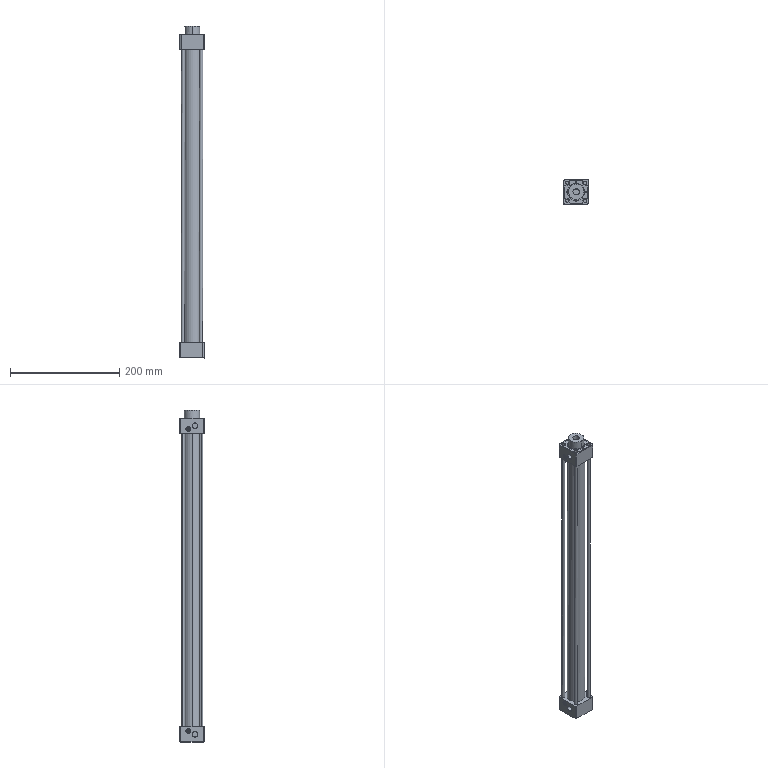Component | SolidWorks | RobotArmTelescopicCylinderSC32x500-1_RobotArmTelescopicCylinderBody-1 | 1 solid | 228 faces | box 45.64 x 45 x 608.04 mm | volume 543651 mm3 | plane 118 | cylinder 102 | cone 8 | commonest cylinder face diameters 6 x24 3.6 x16 31.92 x16 8.4 x16 4.5 x8 3.4 x4 6.8 x4 8 x4